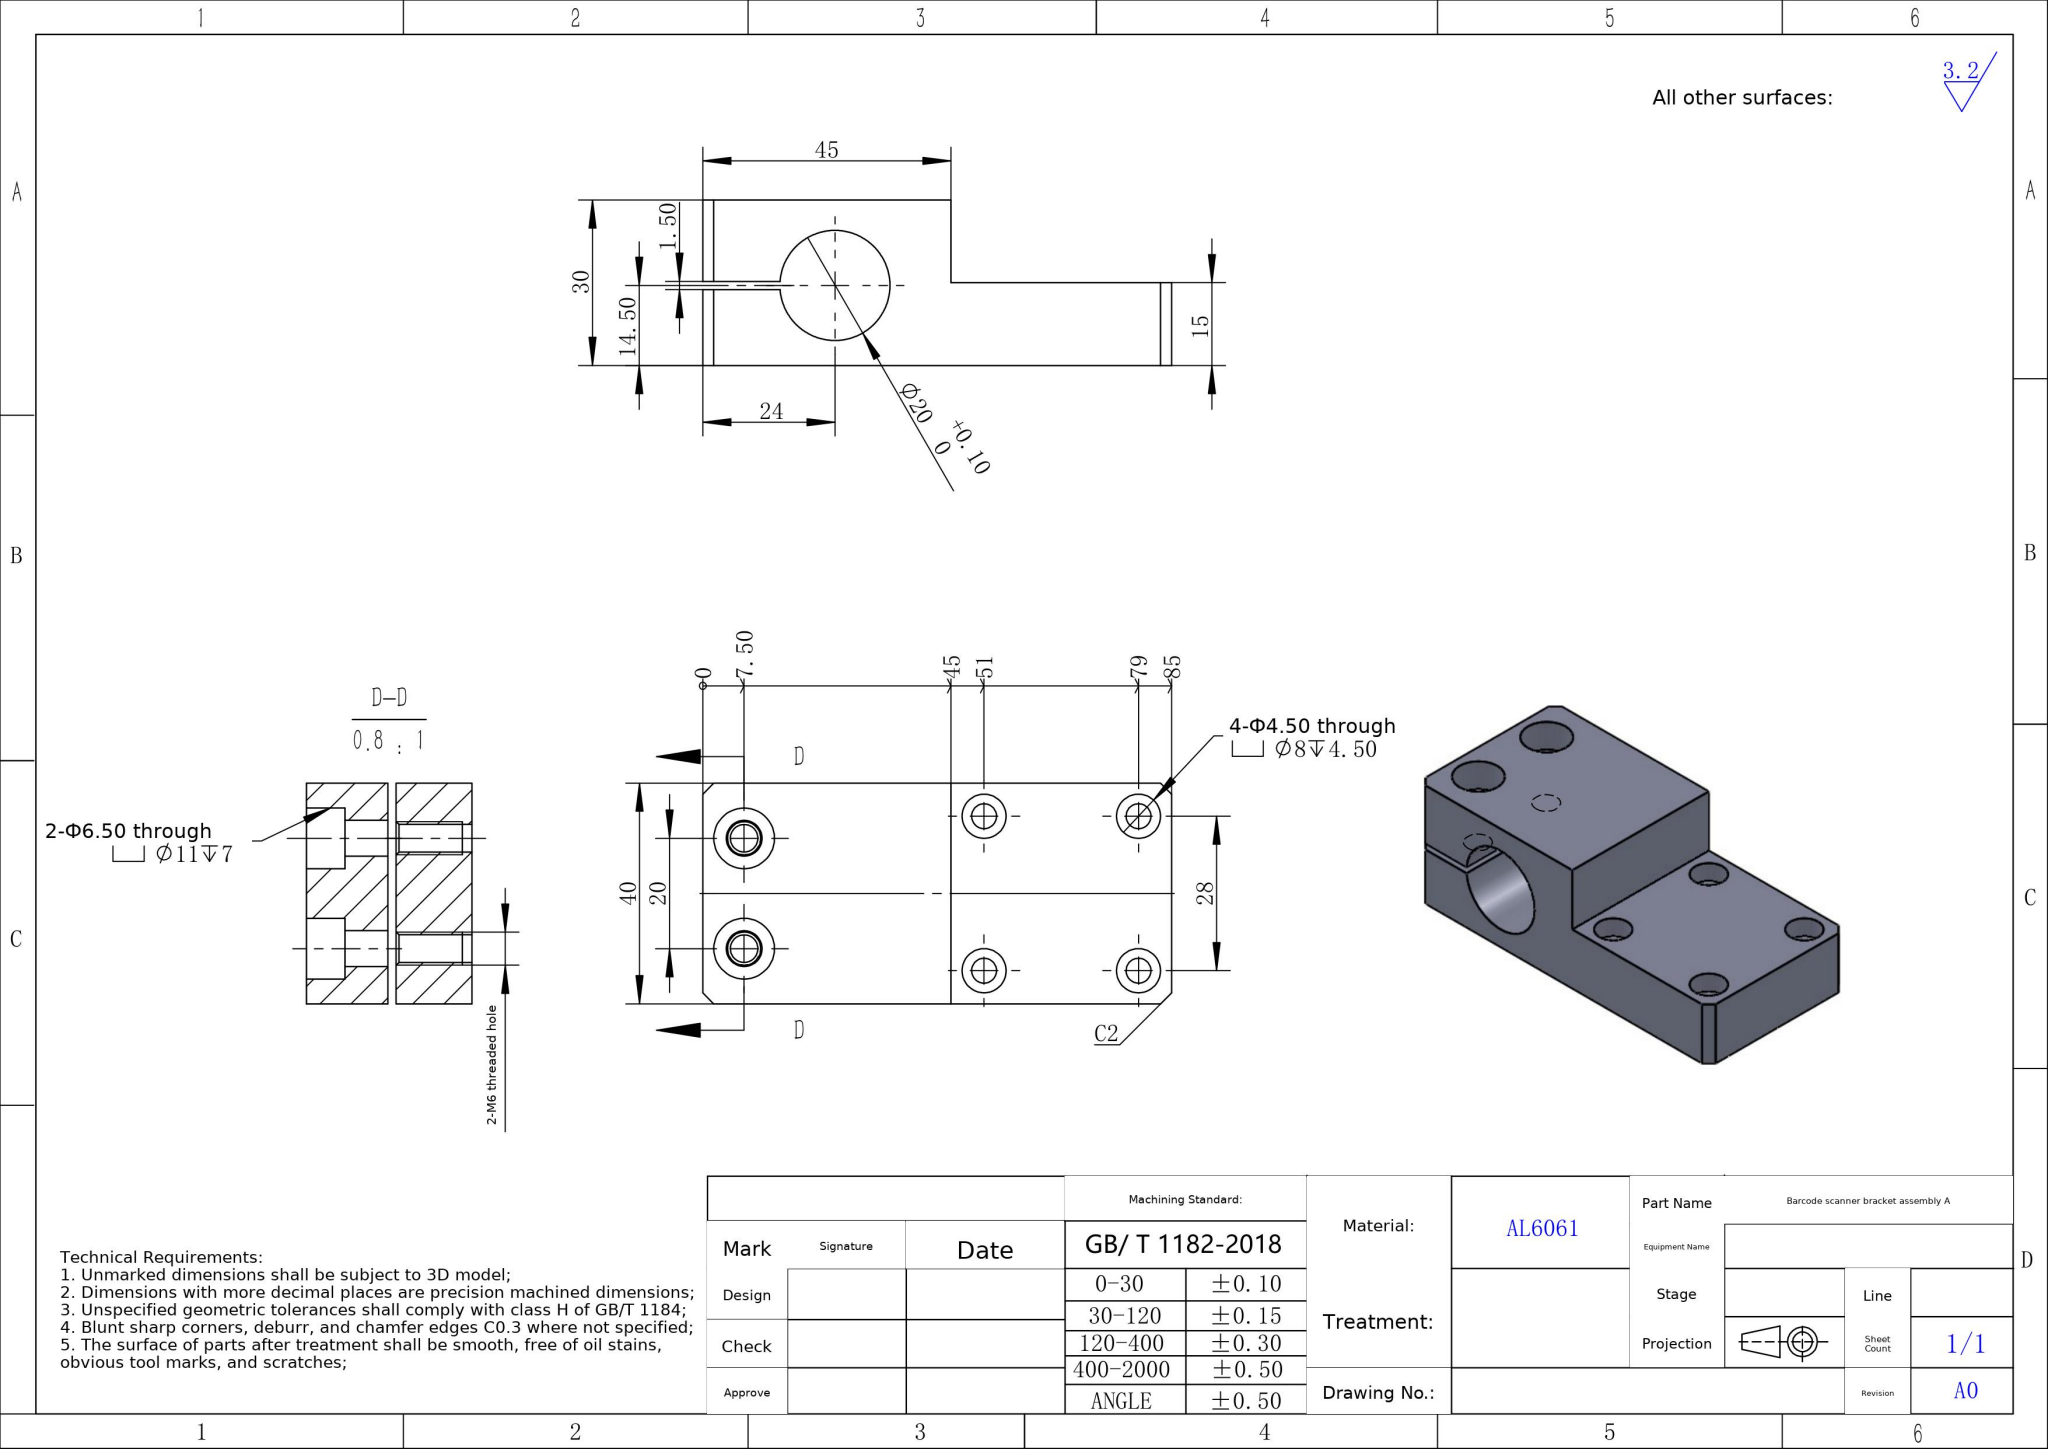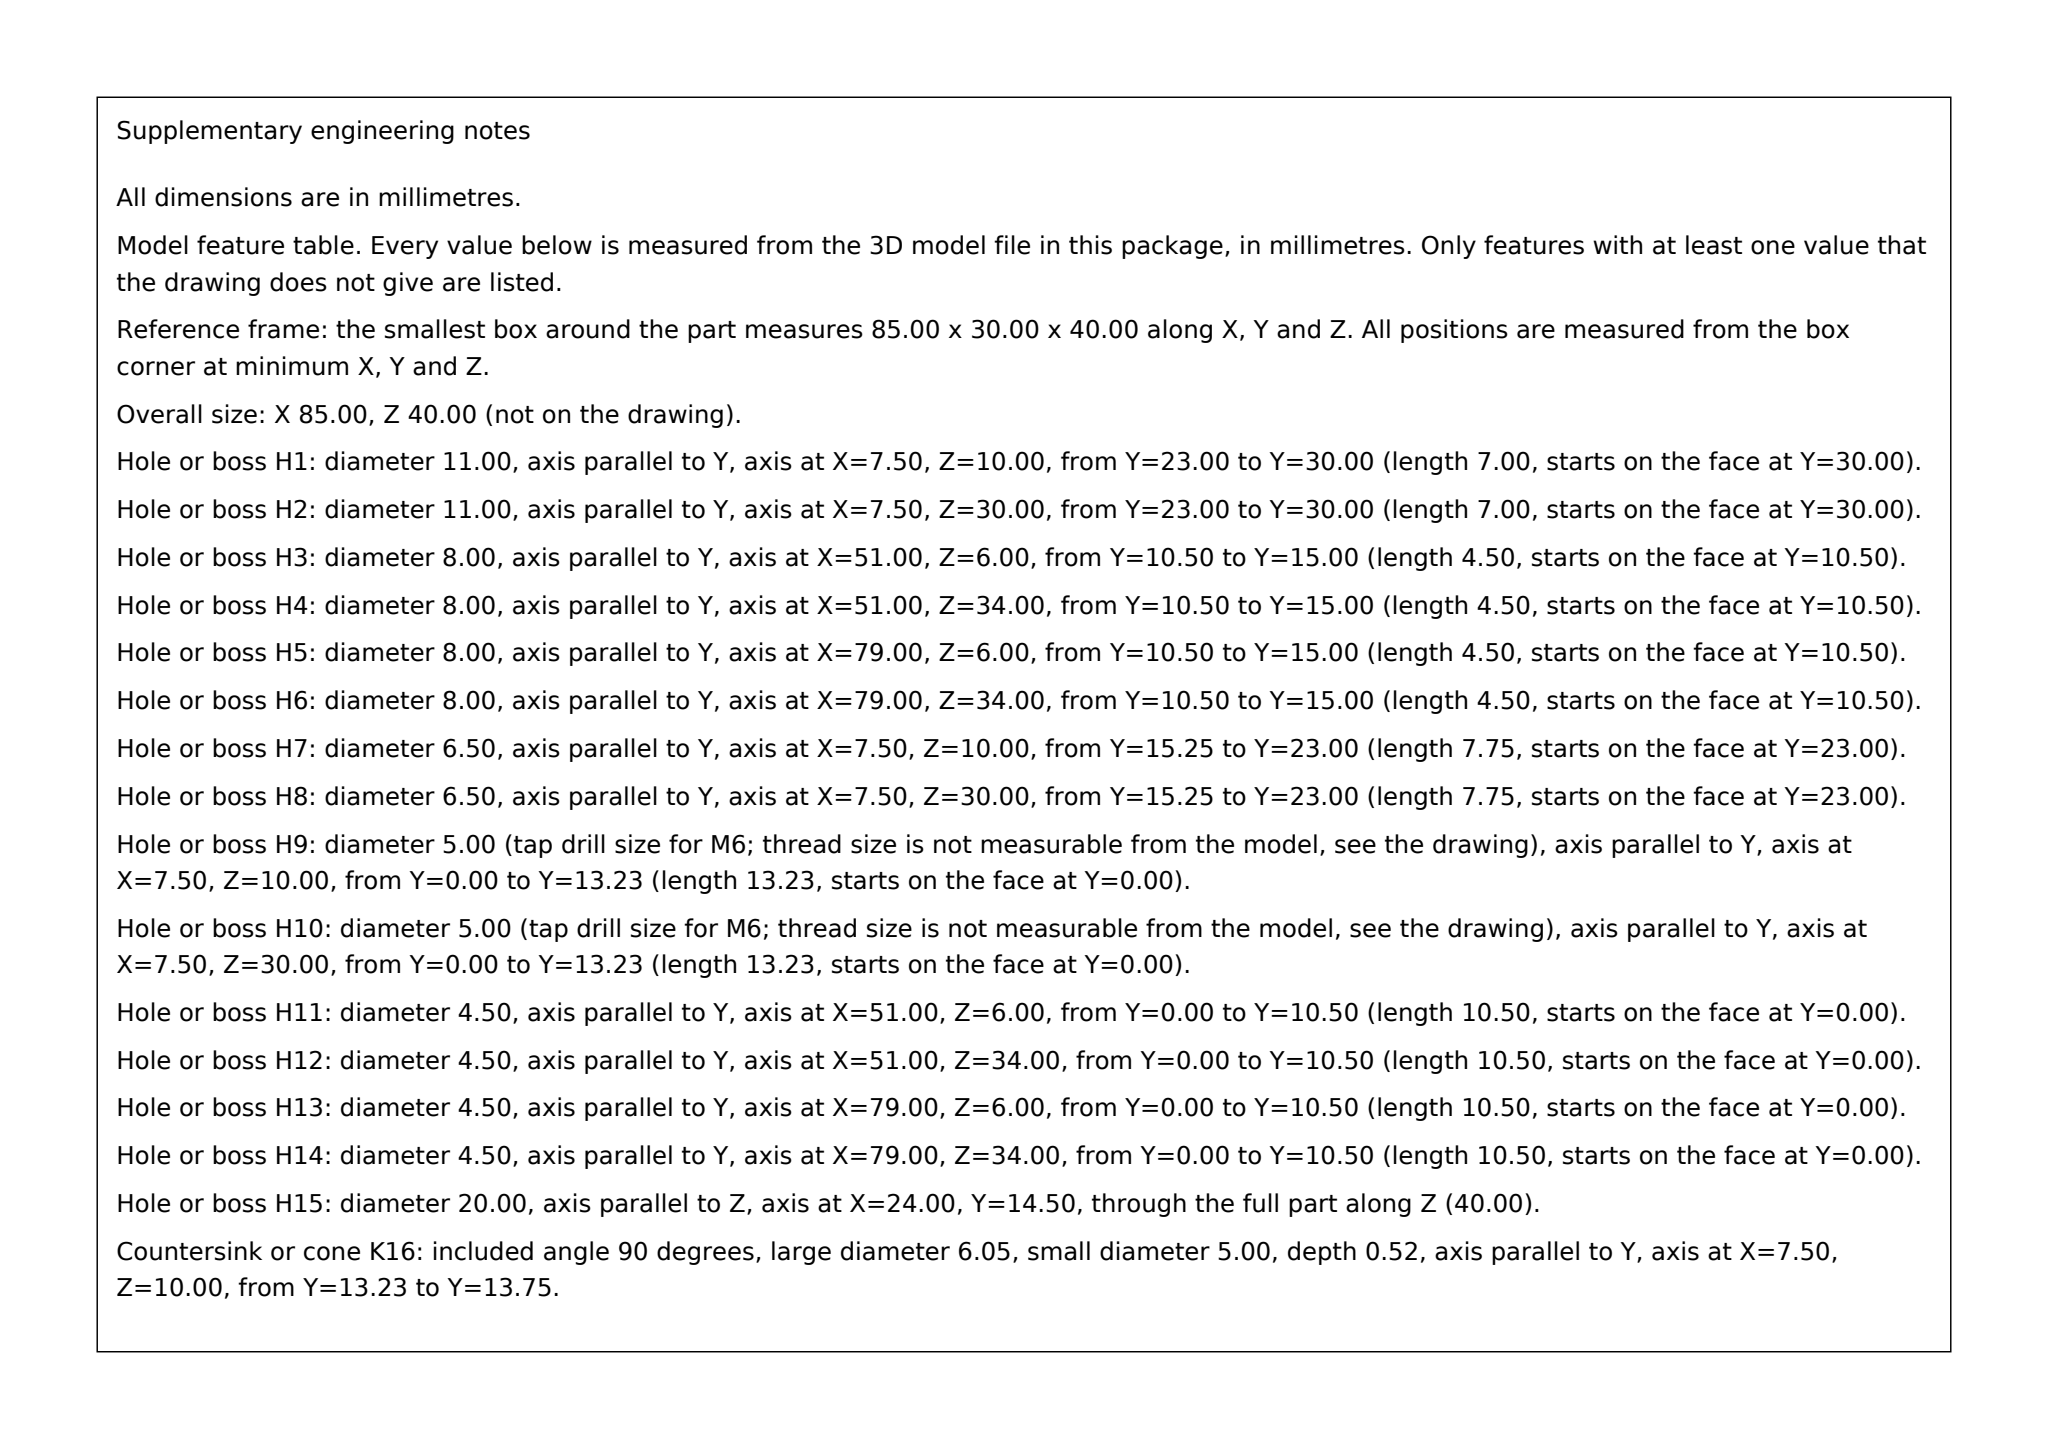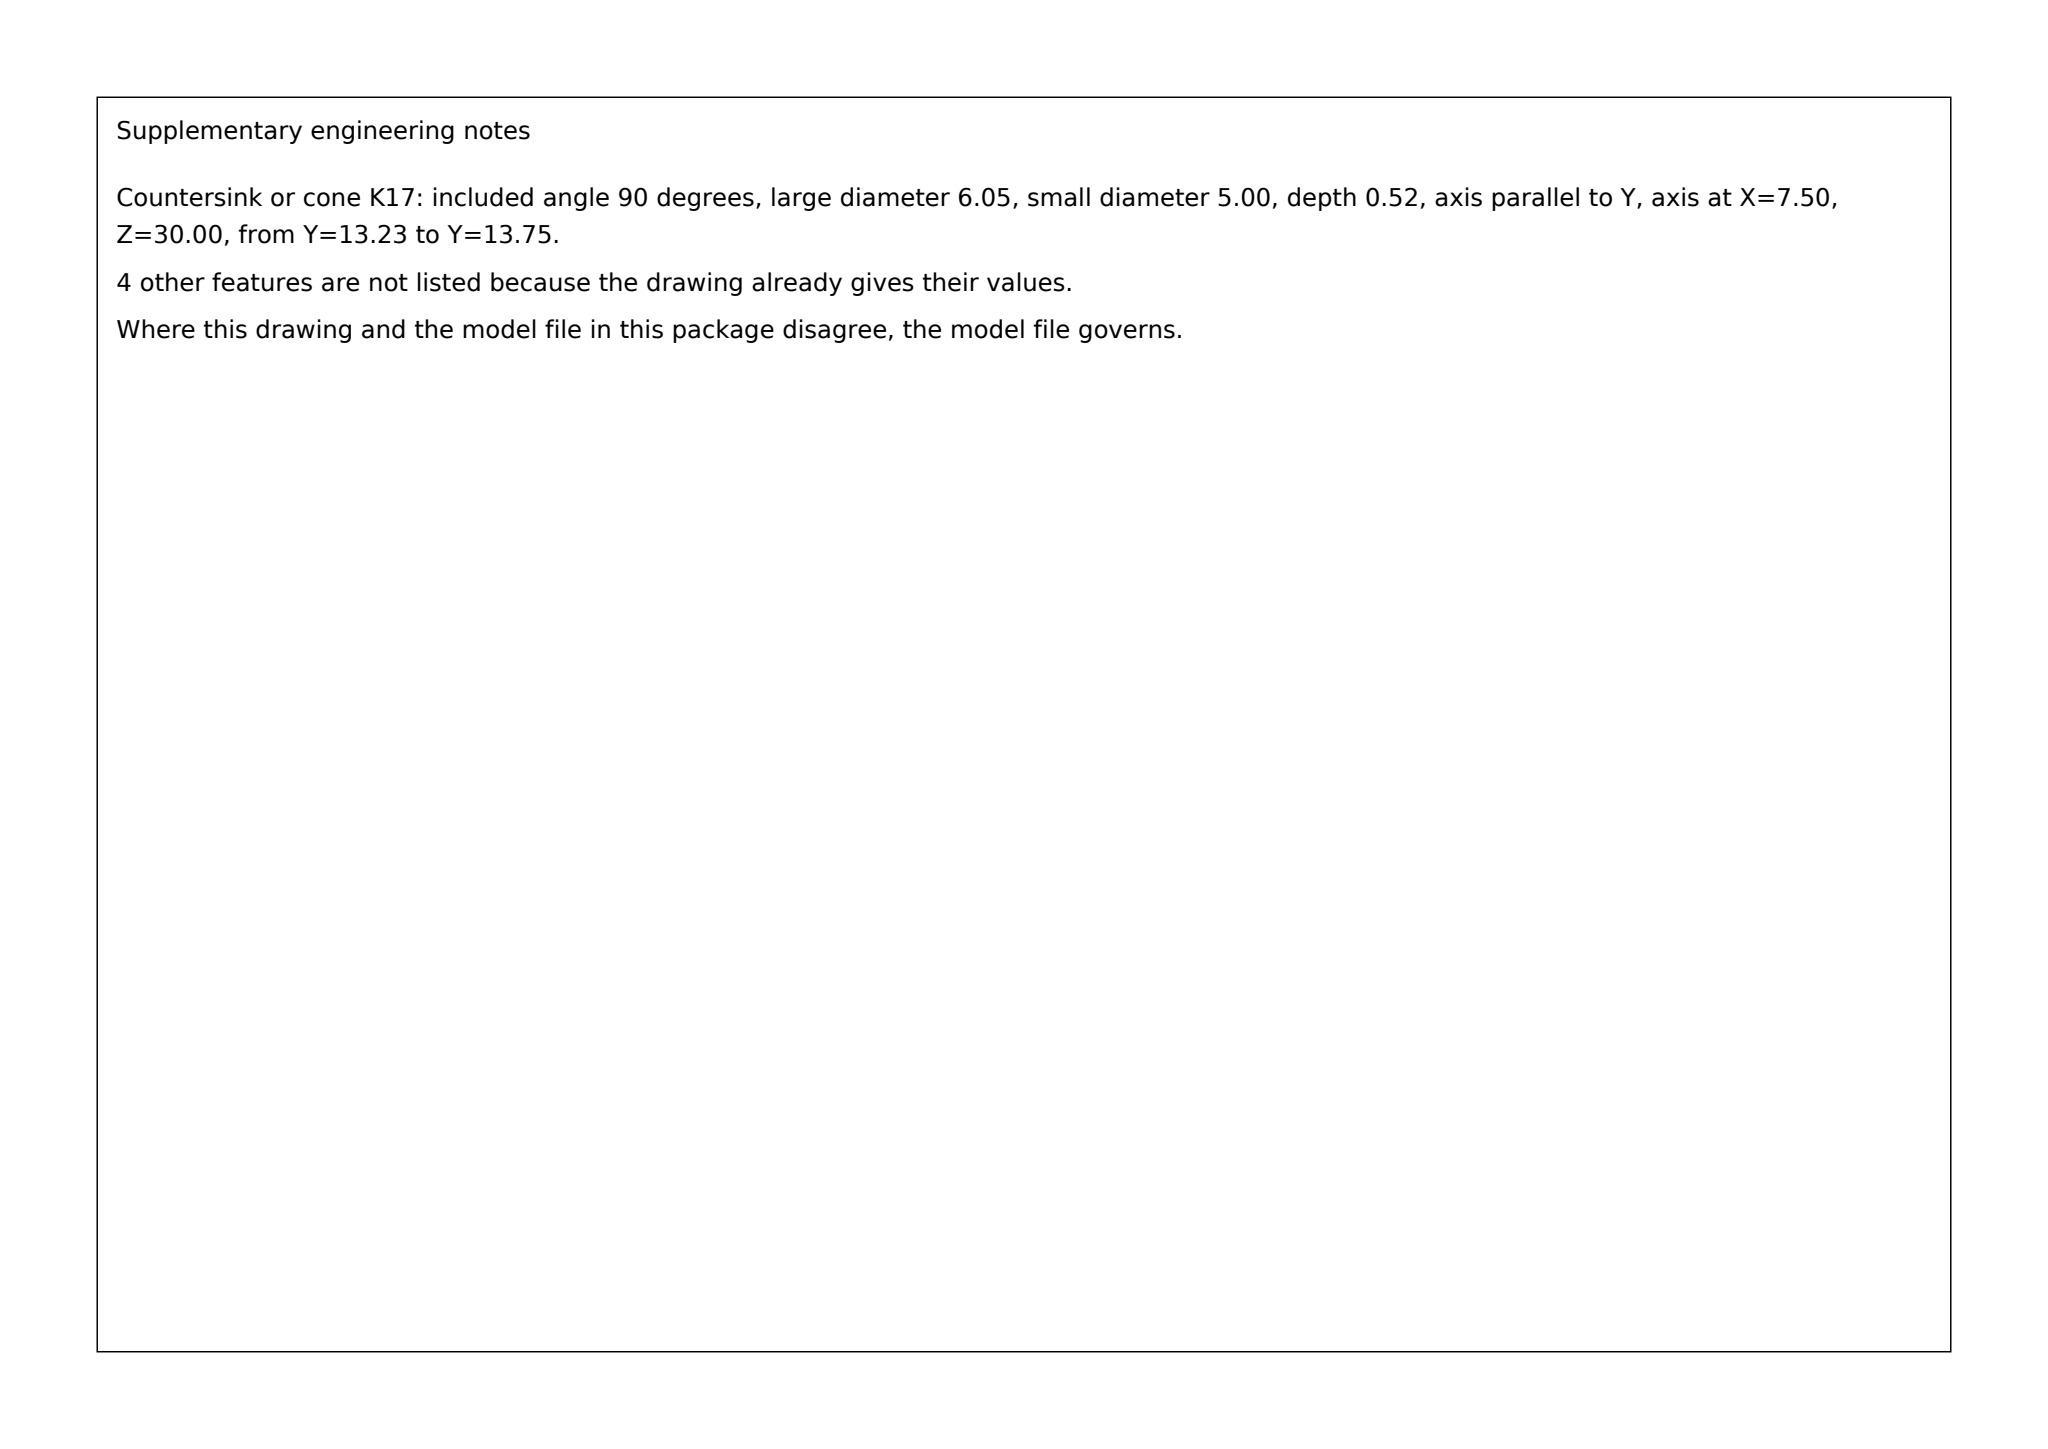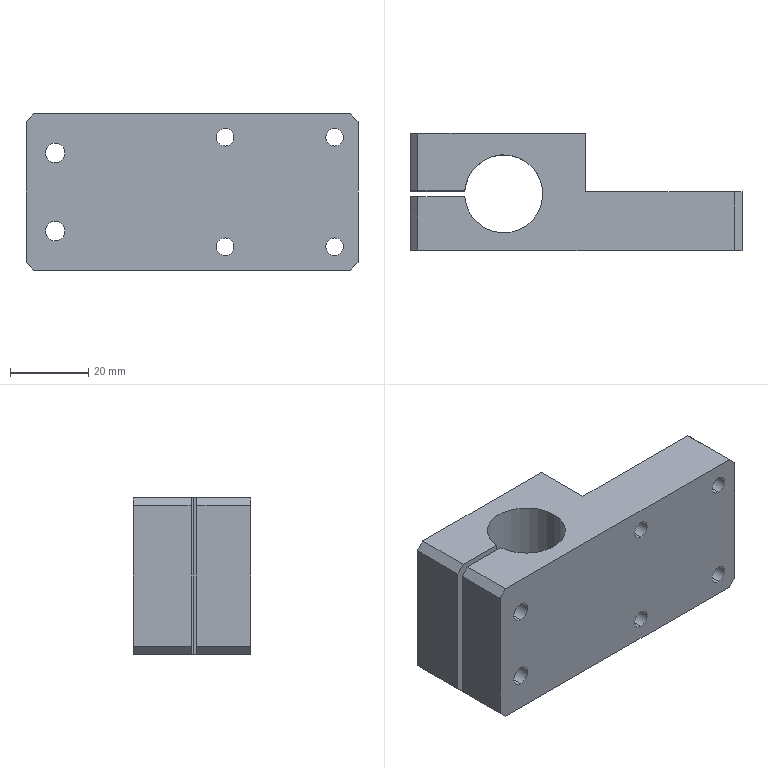Part | SolidWorks | mm | material AL6061 | 1 solid | 57 faces | box 85 x 30 x 40 mm | volume 60457 mm3 | cylinder 30 | plane 23 | cone 4 | commonest cylinder face diameters 8 x8 4.5 x8 5 x4 11 x4 6.5 x4 20 x2